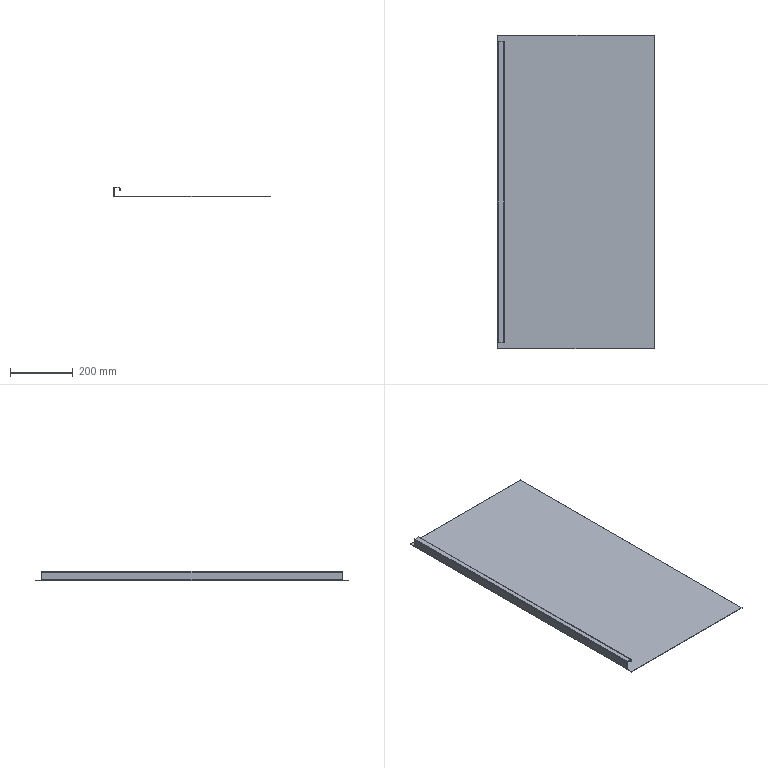Component | SolidWorks | BottomPlate-2 | 1 solid | 38 faces | box 500 x 1000 x 30 mm | volume 826993 mm3 | plane 32 | cylinder 6 | commonest cylinder face diameters 4.473 x2 1.473 x2 5 x1 2 x1
STEP:
#1=CARTESIAN_POINT('',(0.6403,28.583,-3.996));
#2=VERTEX_POINT('',#1);
#3=CARTESIAN_POINT('',(0.6403,28.583,-3.937));
#4=VERTEX_POINT('',#3);
#5=CARTESIAN_POINT('',(0.6403,28.583,-3.996));
#6=DIRECTION('',(0.,0.,1.));
#7=VECTOR('',#6,39.37);
#8=LINE('',#5,#7);
#9=EDGE_CURVE('',#2,#4,#8,.T.);
#10=ORIENTED_EDGE('',*,*,#9,.F.);
#11=CARTESIAN_POINT('',(0.029,28.583,-3.996));
#12=VERTEX_POINT('',#11);
#13=CARTESIAN_POINT('',(-0.,28.583,-3.996));
#14=DIRECTION('',(-1.,-0.,0.));
#15=VECTOR('',#14,39.37);
#16=LINE('',#13,#15);
#17=EDGE_CURVE('',#2,#12,#16,.T.);
#18=ORIENTED_EDGE('',*,*,#17,.T.);
#19=CARTESIAN_POINT('',(0.029,28.583,-3.937));
#20=VERTEX_POINT('',#19);
#21=CARTESIAN_POINT('',(0.029,28.583,-3.937));
#22=DIRECTION('',(0.,-0.,1.));
#23=VECTOR('',#22,39.37);
#24=LINE('',#21,#23);
#25=EDGE_CURVE('',#12,#20,#24,.T.);
#26=ORIENTED_EDGE('',*,*,#25,.T.);
#27=CARTESIAN_POINT('',(9.783,28.583,-3.937));
#28=DIRECTION('',(-1.,-0.,0.));
#29=VECTOR('',#28,39.37);
#30=LINE('',#27,#29);
#31=EDGE_CURVE('',#4,#20,#30,.T.);
#32=ORIENTED_EDGE('',*,*,#31,.F.);
#33=EDGE_LOOP('',(#10,#18,#26,#32));
#34=FACE_OUTER_BOUND('',#33,.T.);
#35=CARTESIAN_POINT('',(-0.,28.583,-3.937));
#36=DIRECTION('',(0.,-1.,-0.));
#37=DIRECTION('',(0.,-0.,1.));
#38=AXIS2_PLACEMENT_3D('',#35,#36,#37);
#39=PLANE('',#38);
#40=ADVANCED_FACE('',(#34),#39,.F.);
#41=CARTESIAN_POINT('',(0.6403,-9.213,-3.996));
#42=VERTEX_POINT('',#41);
#43=CARTESIAN_POINT('',(0.6403,-9.213,-3.937));
#44=VERTEX_POINT('',#43);
#45=CARTESIAN_POINT('',(0.6403,-9.213,-3.996));
#46=DIRECTION('',(0.,-0.,1.));
#47=VECTOR('',#46,39.37);
#48=LINE('',#45,#47);
#49=EDGE_CURVE('',#42,#44,#48,.T.);
#50=ORIENTED_EDGE('',*,*,#49,.T.);
#51=CARTESIAN_POINT('',(0.029,-9.213,-3.937));
#52=VERTEX_POINT('',#51);
#53=CARTESIAN_POINT('',(9.783,-9.213,-3.937));
#54=DIRECTION('',(1.,0.,-0.));
#55=VECTOR('',#54,39.37);
#56=LINE('',#53,#55);
#57=EDGE_CURVE('',#52,#44,#56,.T.);
#58=ORIENTED_EDGE('',*,*,#57,.F.);
#59=CARTESIAN_POINT('',(0.029,-9.213,-3.996));
#60=VERTEX_POINT('',#59);
#61=CARTESIAN_POINT('',(0.029,-9.213,-3.996));
#62=DIRECTION('',(0.,-0.,1.));
#63=VECTOR('',#62,39.37);
#64=LINE('',#61,#63);
#65=EDGE_CURVE('',#60,#52,#64,.T.);
#66=ORIENTED_EDGE('',*,*,#65,.F.);
#67=CARTESIAN_POINT('',(0.7283,-9.213,-3.996));
#68=DIRECTION('',(1.,0.,-0.));
#69=VECTOR('',#68,39.37);
#70=LINE('',#67,#69);
#71=EDGE_CURVE('',#60,#42,#70,.T.);
#72=ORIENTED_EDGE('',*,*,#71,.T.);
#73=EDGE_LOOP('',(#50,#58,#66,#72));
#74=FACE_OUTER_BOUND('',#73,.T.);
#75=CARTESIAN_POINT('',(0.7283,-9.213,-3.937));
#76=DIRECTION('',(-0.,1.,0.));
#77=DIRECTION('',(-0.,0.,-1.));
#78=AXIS2_PLACEMENT_3D('',#75,#76,#77);
#79=PLANE('',#78);
#80=ADVANCED_FACE('',(#74),#79,.F.);
#81=CARTESIAN_POINT('',(0.6403,-9.213,-3.937));
#82=DIRECTION('',(-0.,1.,0.));
#83=VECTOR('',#82,39.37);
#84=LINE('',#81,#83);
#85=EDGE_CURVE('',#44,#4,#84,.T.);
#86=ORIENTED_EDGE('',*,*,#85,.T.);
#87=ORIENTED_EDGE('',*,*,#31,.T.);
#88=CARTESIAN_POINT('',(0.029,28.583,-3.937));
#89=DIRECTION('',(-0.,1.,0.));
#90=VECTOR('',#89,39.37);
#91=LINE('',#88,#90);
#92=EDGE_CURVE('',#52,#20,#91,.T.);
#93=ORIENTED_EDGE('',*,*,#92,.F.);
#94=ORIENTED_EDGE('',*,*,#57,.T.);
#95=EDGE_LOOP('',(#86,#87,#93,#94));
#96=FACE_OUTER_BOUND('',#95,.T.);
#97=CARTESIAN_POINT('',(9.783,9.685,-3.937));
#98=DIRECTION('',(-0.,0.,-1.));
#99=DIRECTION('',(-1.,-0.,0.));
#100=AXIS2_PLACEMENT_3D('',#97,#98,#99);
#101=PLANE('',#100);
#102=ADVANCED_FACE('',(#96),#101,.F.);
#103=ORIENTED_EDGE('',*,*,#17,.F.);
#104=CARTESIAN_POINT('',(0.6403,-9.213,-3.996));
#105=DIRECTION('',(-0.,1.,0.));
#106=VECTOR('',#105,39.37);
#107=LINE('',#104,#106);
#108=EDGE_CURVE('',#42,#2,#107,.T.);
#109=ORIENTED_EDGE('',*,*,#108,.F.);
#110=ORIENTED_EDGE('',*,*,#71,.F.);
#111=CARTESIAN_POINT('',(0.029,28.583,-3.996));
#112=DIRECTION('',(0.,-1.,-0.));
#113=VECTOR('',#112,39.37);
#114=LINE('',#111,#113);
#115=EDGE_CURVE('',#12,#60,#114,.T.);
#116=ORIENTED_EDGE('',*,*,#115,.F.);
#117=EDGE_LOOP('',(#103,#109,#110,#116));
#118=FACE_OUTER_BOUND('',#117,.T.);
#119=CARTESIAN_POINT('',(9.783,9.685,-3.996));
#120=DIRECTION('',(-0.,0.,-1.));
#121=DIRECTION('',(-1.,-0.,0.));
#122=AXIS2_PLACEMENT_3D('',#119,#120,#121);
#123=PLANE('',#122);
#124=ADVANCED_FACE('',(#118),#123,.T.);
#125=CARTESIAN_POINT('',(0.,-9.213,-4.025));
#126=VERTEX_POINT('',#125);
#127=CARTESIAN_POINT('',(0.,-9.213,-5.02));
#128=VERTEX_POINT('',#127);
#129=CARTESIAN_POINT('',(0.,-9.213,-5.118));
#130=DIRECTION('',(-0.,-0.,-1.));
#131=VECTOR('',#130,39.37);
#132=LINE('',#129,#131);
#133=EDGE_CURVE('',#126,#128,#132,.T.);
#134=ORIENTED_EDGE('',*,*,#133,.F.);
#135=CARTESIAN_POINT('',(-0.05906,-9.213,-4.025));
#136=VERTEX_POINT('',#135);
#137=CARTESIAN_POINT('',(0.,-9.213,-4.025));
#138=DIRECTION('',(-1.,-0.,-0.));
#139=VECTOR('',#138,39.37);
#140=LINE('',#137,#139);
#141=EDGE_CURVE('',#126,#136,#140,.T.);
#142=ORIENTED_EDGE('',*,*,#141,.T.);
#143=CARTESIAN_POINT('',(-0.05906,-9.213,-5.02));
#144=VERTEX_POINT('',#143);
#145=CARTESIAN_POINT('',(-0.05906,-9.213,-3.937));
#146=DIRECTION('',(-0.,-0.,-1.));
#147=VECTOR('',#146,39.37);
#148=LINE('',#145,#147);
#149=EDGE_CURVE('',#136,#144,#148,.T.);
#150=ORIENTED_EDGE('',*,*,#149,.T.);
#151=CARTESIAN_POINT('',(0.,-9.213,-5.02));
#152=DIRECTION('',(-1.,-0.,0.));
#153=VECTOR('',#152,39.37);
#154=LINE('',#151,#153);
#155=EDGE_CURVE('',#128,#144,#154,.T.);
#156=ORIENTED_EDGE('',*,*,#155,.F.);
#157=EDGE_LOOP('',(#134,#142,#150,#156));
#158=FACE_OUTER_BOUND('',#157,.T.);
#159=CARTESIAN_POINT('',(-0.05906,-9.213,-3.937));
#160=DIRECTION('',(0.,-1.,0.));
#161=DIRECTION('',(-1.,-0.,0.));
#162=AXIS2_PLACEMENT_3D('',#159,#160,#161);
#163=PLANE('',#162);
#164=ADVANCED_FACE('',(#158),#163,.T.);
#165=CARTESIAN_POINT('',(-0.05906,28.583,-4.025));
#166=VERTEX_POINT('',#165);
#167=CARTESIAN_POINT('',(-0.05906,-9.213,-4.025));
#168=DIRECTION('',(-0.,1.,-0.));
#169=VECTOR('',#168,39.37);
#170=LINE('',#167,#169);
#171=EDGE_CURVE('',#136,#166,#170,.T.);
#172=ORIENTED_EDGE('',*,*,#171,.T.);
#173=CARTESIAN_POINT('',(-0.05906,28.583,-5.02));
#174=VERTEX_POINT('',#173);
#175=CARTESIAN_POINT('',(-0.05906,28.583,-5.059));
#176=DIRECTION('',(0.,0.,1.));
#177=VECTOR('',#176,39.37);
#178=LINE('',#175,#177);
#179=EDGE_CURVE('',#174,#166,#178,.T.);
#180=ORIENTED_EDGE('',*,*,#179,.F.);
#181=CARTESIAN_POINT('',(-0.05906,28.583,-5.02));
#182=DIRECTION('',(-0.,1.,-0.));
#183=VECTOR('',#182,39.37);
#184=LINE('',#181,#183);
#185=EDGE_CURVE('',#144,#174,#184,.T.);
#186=ORIENTED_EDGE('',*,*,#185,.F.);
#187=ORIENTED_EDGE('',*,*,#149,.F.);
#188=EDGE_LOOP('',(#172,#180,#186,#187));
#189=FACE_OUTER_BOUND('',#188,.T.);
#190=CARTESIAN_POINT('',(-0.05906,9.685,-5.118));
#191=DIRECTION('',(1.,0.,-0.));
#192=DIRECTION('',(-0.,-0.,-1.));
#193=AXIS2_PLACEMENT_3D('',#190,#191,#192);
#194=PLANE('',#193);
#195=ADVANCED_FACE('',(#189),#194,.F.);
#196=CARTESIAN_POINT('',(-0.,28.583,-5.02));
#197=VERTEX_POINT('',#196);
#198=CARTESIAN_POINT('',(-0.,28.583,-4.025));
#199=VERTEX_POINT('',#198);
#200=CARTESIAN_POINT('',(-0.,28.583,-5.118));
#201=DIRECTION('',(0.,0.,1.));
#202=VECTOR('',#201,39.37);
#203=LINE('',#200,#202);
#204=EDGE_CURVE('',#197,#199,#203,.T.);
#205=ORIENTED_EDGE('',*,*,#204,.T.);
#206=CARTESIAN_POINT('',(0.,-9.213,-4.025));
#207=DIRECTION('',(-0.,1.,-0.));
#208=VECTOR('',#207,39.37);
#209=LINE('',#206,#208);
#210=EDGE_CURVE('',#126,#199,#209,.T.);
#211=ORIENTED_EDGE('',*,*,#210,.F.);
#212=ORIENTED_EDGE('',*,*,#133,.T.);
#213=CARTESIAN_POINT('',(-0.,28.583,-5.02));
#214=DIRECTION('',(0.,-1.,0.));
#215=VECTOR('',#214,39.37);
#216=LINE('',#213,#215);
#217=EDGE_CURVE('',#197,#128,#216,.T.);
#218=ORIENTED_EDGE('',*,*,#217,.F.);
#219=EDGE_LOOP('',(#205,#211,#212,#218));
#220=FACE_OUTER_BOUND('',#219,.T.);
#221=CARTESIAN_POINT('',(-0.,9.685,-5.118));
#222=DIRECTION('',(1.,0.,-0.));
#223=DIRECTION('',(-0.,-0.,-1.));
#224=AXIS2_PLACEMENT_3D('',#221,#222,#223);
#225=PLANE('',#224);
#226=ADVANCED_FACE('',(#220),#225,.T.);
#227=CARTESIAN_POINT('',(-0.05906,-10.,-5.059));
#228=VERTEX_POINT('',#227);
#229=CARTESIAN_POINT('',(-0.05906,-9.242,-5.059));
#230=VERTEX_POINT('',#229);
#231=CARTESIAN_POINT('',(-0.05906,-10.,-5.059));
#232=DIRECTION('',(-0.,1.,-0.));
#233=VECTOR('',#232,39.37);
#234=LINE('',#231,#233);
#235=EDGE_CURVE('',#228,#230,#234,.T.);
#236=ORIENTED_EDGE('',*,*,#235,.T.);
#237=CARTESIAN_POINT('',(-0.05906,-9.242,-5.118));
#238=VERTEX_POINT('',#237);
#239=CARTESIAN_POINT('',(-0.05906,-9.242,-5.059));
#240=DIRECTION('',(-0.,-0.,-1.));
#241=VECTOR('',#240,39.37);
#242=LINE('',#239,#241);
#243=EDGE_CURVE('',#230,#238,#242,.T.);
#244=ORIENTED_EDGE('',*,*,#243,.T.);
#245=CARTESIAN_POINT('',(-0.05906,-10.,-5.118));
#246=VERTEX_POINT('',#245);
#247=CARTESIAN_POINT('',(-0.05906,-10.,-5.118));
#248=DIRECTION('',(-0.,1.,-0.));
#249=VECTOR('',#248,39.37);
#250=LINE('',#247,#249);
#251=EDGE_CURVE('',#246,#238,#250,.T.);
#252=ORIENTED_EDGE('',*,*,#251,.F.);
#253=CARTESIAN_POINT('',(-0.05906,-10.,-5.059));
#254=DIRECTION('',(-0.,-0.,-1.));
#255=VECTOR('',#254,39.37);
#256=LINE('',#253,#255);
#257=EDGE_CURVE('',#228,#246,#256,.T.);
#258=ORIENTED_EDGE('',*,*,#257,.F.);
#259=EDGE_LOOP('',(#236,#244,#252,#258));
#260=FACE_OUTER_BOUND('',#259,.T.);
#261=CARTESIAN_POINT('',(-0.05906,-10.,-5.059));
#262=DIRECTION('',(-1.,-0.,0.));
#263=DIRECTION('',(-0.,1.,-0.));
#264=AXIS2_PLACEMENT_3D('',#261,#262,#263);
#265=PLANE('',#264);
#266=ADVANCED_FACE('',(#260),#265,.T.);
#267=CARTESIAN_POINT('',(-0.05906,28.612,-5.118));
#268=VERTEX_POINT('',#267);
#269=CARTESIAN_POINT('',(-0.05906,29.37,-5.118));
#270=VERTEX_POINT('',#269);
#271=CARTESIAN_POINT('',(-0.05906,-10.,-5.118));
#272=DIRECTION('',(-0.,1.,-0.));
#273=VECTOR('',#272,39.37);
#274=LINE('',#271,#273);
#275=EDGE_CURVE('',#268,#270,#274,.T.);
#276=ORIENTED_EDGE('',*,*,#275,.F.);
#277=CARTESIAN_POINT('',(-0.05906,28.612,-5.059));
#278=VERTEX_POINT('',#277);
#279=CARTESIAN_POINT('',(-0.05906,28.612,-5.059));
#280=DIRECTION('',(-0.,-0.,-1.));
#281=VECTOR('',#280,39.37);
#282=LINE('',#279,#281);
#283=EDGE_CURVE('',#278,#268,#282,.T.);
#284=ORIENTED_EDGE('',*,*,#283,.F.);
#285=CARTESIAN_POINT('',(-0.05906,29.37,-5.059));
#286=VERTEX_POINT('',#285);
#287=CARTESIAN_POINT('',(-0.05906,-10.,-5.059));
#288=DIRECTION('',(-0.,1.,-0.));
#289=VECTOR('',#288,39.37);
#290=LINE('',#287,#289);
#291=EDGE_CURVE('',#278,#286,#290,.T.);
#292=ORIENTED_EDGE('',*,*,#291,.T.);
#293=CARTESIAN_POINT('',(-0.05906,29.37,-5.059));
#294=DIRECTION('',(-0.,-0.,-1.));
#295=VECTOR('',#294,39.37);
#296=LINE('',#293,#295);
#297=EDGE_CURVE('',#286,#270,#296,.T.);
#298=ORIENTED_EDGE('',*,*,#297,.T.);
#299=EDGE_LOOP('',(#276,#284,#292,#298));
#300=FACE_OUTER_BOUND('',#299,.T.);
#301=CARTESIAN_POINT('',(-0.05906,-10.,-5.059));
#302=DIRECTION('',(-1.,-0.,0.));
#303=DIRECTION('',(-0.,1.,-0.));
#304=AXIS2_PLACEMENT_3D('',#301,#302,#303);
#305=PLANE('',#304);
#306=ADVANCED_FACE('',(#300),#305,.T.);
#307=CARTESIAN_POINT('',(0.0689,-9.242,-5.059));
#308=VERTEX_POINT('',#307);
#309=CARTESIAN_POINT('',(-0.05906,-9.242,-5.059));
#310=DIRECTION('',(1.,0.,-0.));
#311=VECTOR('',#310,39.37);
#312=LINE('',#309,#311);
#313=EDGE_CURVE('',#230,#308,#312,.T.);
#314=ORIENTED_EDGE('',*,*,#313,.F.);
#315=ORIENTED_EDGE('',*,*,#235,.F.);
#316=CARTESIAN_POINT('',(19.626,-10.,-5.059));
#317=VERTEX_POINT('',#316);
#318=CARTESIAN_POINT('',(19.626,-10.,-5.059));
#319=DIRECTION('',(-1.,-0.,0.));
#320=VECTOR('',#319,39.37);
#321=LINE('',#318,#320);
#322=EDGE_CURVE('',#317,#228,#321,.T.);
#323=ORIENTED_EDGE('',*,*,#322,.F.);
#324=CARTESIAN_POINT('',(19.626,29.37,-5.059));
#325=VERTEX_POINT('',#324);
#326=CARTESIAN_POINT('',(19.626,-10.,-5.059));
#327=DIRECTION('',(0.,-1.,0.));
#328=VECTOR('',#327,39.37);
#329=LINE('',#326,#328);
#330=EDGE_CURVE('',#325,#317,#329,.T.);
#331=ORIENTED_EDGE('',*,*,#330,.F.);
#332=CARTESIAN_POINT('',(19.626,29.37,-5.059));
#333=DIRECTION('',(1.,0.,-0.));
#334=VECTOR('',#333,39.37);
#335=LINE('',#332,#334);
#336=EDGE_CURVE('',#286,#325,#335,.T.);
#337=ORIENTED_EDGE('',*,*,#336,.F.);
#338=ORIENTED_EDGE('',*,*,#291,.F.);
#339=CARTESIAN_POINT('',(0.0689,28.612,-5.059));
#340=VERTEX_POINT('',#339);
#341=CARTESIAN_POINT('',(0.0689,28.612,-5.059));
#342=DIRECTION('',(-1.,0.,0.));
#343=VECTOR('',#342,39.37);
#344=LINE('',#341,#343);
#345=EDGE_CURVE('',#340,#278,#344,.T.);
#346=ORIENTED_EDGE('',*,*,#345,.F.);
#347=CARTESIAN_POINT('',(0.0689,28.583,-5.059));
#348=VERTEX_POINT('',#347);
#349=CARTESIAN_POINT('',(0.0689,28.583,-5.059));
#350=DIRECTION('',(-0.,1.,-0.));
#351=VECTOR('',#350,39.37);
#352=LINE('',#349,#351);
#353=EDGE_CURVE('',#348,#340,#352,.T.);
#354=ORIENTED_EDGE('',*,*,#353,.F.);
#355=CARTESIAN_POINT('',(0.03937,28.583,-5.059));
#356=VERTEX_POINT('',#355);
#357=CARTESIAN_POINT('',(0.03937,28.583,-5.059));
#358=DIRECTION('',(1.,0.,-0.));
#359=VECTOR('',#358,39.37);
#360=LINE('',#357,#359);
#361=EDGE_CURVE('',#356,#348,#360,.T.);
#362=ORIENTED_EDGE('',*,*,#361,.F.);
#363=CARTESIAN_POINT('',(0.03937,-9.213,-5.059));
#364=VERTEX_POINT('',#363);
#365=CARTESIAN_POINT('',(0.03937,-9.213,-5.059));
#366=DIRECTION('',(-0.,1.,-0.));
#367=VECTOR('',#366,39.37);
#368=LINE('',#365,#367);
#369=EDGE_CURVE('',#364,#356,#368,.T.);
#370=ORIENTED_EDGE('',*,*,#369,.F.);
#371=CARTESIAN_POINT('',(0.0689,-9.213,-5.059));
#372=VERTEX_POINT('',#371);
#373=CARTESIAN_POINT('',(0.0689,-9.213,-5.059));
#374=DIRECTION('',(-1.,-0.,0.));
#375=VECTOR('',#374,39.37);
#376=LINE('',#373,#375);
#377=EDGE_CURVE('',#372,#364,#376,.T.);
#378=ORIENTED_EDGE('',*,*,#377,.F.);
#379=CARTESIAN_POINT('',(0.0689,-9.242,-5.059));
#380=DIRECTION('',(-0.,1.,-0.));
#381=VECTOR('',#380,39.37);
#382=LINE('',#379,#381);
#383=EDGE_CURVE('',#308,#372,#382,.T.);
#384=ORIENTED_EDGE('',*,*,#383,.F.);
#385=EDGE_LOOP('',(#314,#315,#323,#331,#337,#338,#346,#354,#362,#370,#378,#384));
#386=FACE_OUTER_BOUND('',#385,.T.);
#387=CARTESIAN_POINT('',(9.783,9.685,-5.059));
#388=DIRECTION('',(-0.,-0.,-1.));
#389=DIRECTION('',(-1.,-0.,0.));
#390=AXIS2_PLACEMENT_3D('',#387,#388,#389);
#391=PLANE('',#390);
#392=ADVANCED_FACE('',(#386),#391,.F.);
#393=ORIENTED_EDGE('',*,*,#251,.T.);
#394=CARTESIAN_POINT('',(0.0689,-9.242,-5.118));
#395=VERTEX_POINT('',#394);
#396=CARTESIAN_POINT('',(9.783,-9.242,-5.118));
#397=DIRECTION('',(1.,0.,-0.));
#398=VECTOR('',#397,39.37);
#399=LINE('',#396,#398);
#400=EDGE_CURVE('',#238,#395,#399,.T.);
#401=ORIENTED_EDGE('',*,*,#400,.T.);
#402=CARTESIAN_POINT('',(0.0689,-9.213,-5.118));
#403=VERTEX_POINT('',#402);
#404=CARTESIAN_POINT('',(0.0689,9.685,-5.118));
#405=DIRECTION('',(-0.,1.,-0.));
#406=VECTOR('',#405,39.37);
#407=LINE('',#404,#406);
#408=EDGE_CURVE('',#395,#403,#407,.T.);
#409=ORIENTED_EDGE('',*,*,#408,.T.);
#410=CARTESIAN_POINT('',(0.03937,-9.213,-5.118));
#411=VERTEX_POINT('',#410);
#412=CARTESIAN_POINT('',(9.783,-9.213,-5.118));
#413=DIRECTION('',(-1.,-0.,0.));
#414=VECTOR('',#413,39.37);
#415=LINE('',#412,#414);
#416=EDGE_CURVE('',#403,#411,#415,.T.);
#417=ORIENTED_EDGE('',*,*,#416,.T.);
#418=CARTESIAN_POINT('',(0.03937,28.583,-5.118));
#419=VERTEX_POINT('',#418);
#420=CARTESIAN_POINT('',(0.03937,-9.213,-5.118));
#421=DIRECTION('',(-0.,1.,-0.));
#422=VECTOR('',#421,39.37);
#423=LINE('',#420,#422);
#424=EDGE_CURVE('',#411,#419,#423,.T.);
#425=ORIENTED_EDGE('',*,*,#424,.T.);
#426=CARTESIAN_POINT('',(0.0689,28.583,-5.118));
#427=VERTEX_POINT('',#426);
#428=CARTESIAN_POINT('',(9.783,28.583,-5.118));
#429=DIRECTION('',(1.,0.,-0.));
#430=VECTOR('',#429,39.37);
#431=LINE('',#428,#430);
#432=EDGE_CURVE('',#419,#427,#431,.T.);
#433=ORIENTED_EDGE('',*,*,#432,.T.);
#434=CARTESIAN_POINT('',(0.0689,28.612,-5.118));
#435=VERTEX_POINT('',#434);
#436=CARTESIAN_POINT('',(0.0689,9.685,-5.118));
#437=DIRECTION('',(-0.,1.,-0.));
#438=VECTOR('',#437,39.37);
#439=LINE('',#436,#438);
#440=EDGE_CURVE('',#427,#435,#439,.T.);
#441=ORIENTED_EDGE('',*,*,#440,.T.);
#442=CARTESIAN_POINT('',(9.783,28.612,-5.118));
#443=DIRECTION('',(-1.,0.,0.));
#444=VECTOR('',#443,39.37);
#445=LINE('',#442,#444);
#446=EDGE_CURVE('',#435,#268,#445,.T.);
#447=ORIENTED_EDGE('',*,*,#446,.T.);
#448=ORIENTED_EDGE('',*,*,#275,.T.);
#449=CARTESIAN_POINT('',(19.626,29.37,-5.118));
#450=VERTEX_POINT('',#449);
#451=CARTESIAN_POINT('',(19.626,29.37,-5.118));
#452=DIRECTION('',(1.,0.,-0.));
#453=VECTOR('',#452,39.37);
#454=LINE('',#451,#453);
#455=EDGE_CURVE('',#270,#450,#454,.T.);
#456=ORIENTED_EDGE('',*,*,#455,.T.);
#457=CARTESIAN_POINT('',(19.626,-10.,-5.118));
#458=VERTEX_POINT('',#457);
#459=CARTESIAN_POINT('',(19.626,-10.,-5.118));
#460=DIRECTION('',(0.,-1.,0.));
#461=VECTOR('',#460,39.37);
#462=LINE('',#459,#461);
#463=EDGE_CURVE('',#450,#458,#462,.T.);
#464=ORIENTED_EDGE('',*,*,#463,.T.);
#465=CARTESIAN_POINT('',(19.626,-10.,-5.118));
#466=DIRECTION('',(-1.,-0.,0.));
#467=VECTOR('',#466,39.37);
#468=LINE('',#465,#467);
#469=EDGE_CURVE('',#458,#246,#468,.T.);
#470=ORIENTED_EDGE('',*,*,#469,.T.);
#471=EDGE_LOOP('',(#393,#401,#409,#417,#425,#433,#441,#447,#448,#456,#464,#470));
#472=FACE_OUTER_BOUND('',#471,.T.);
#473=CARTESIAN_POINT('',(9.783,9.685,-5.118));
#474=DIRECTION('',(-0.,-0.,-1.));
#475=DIRECTION('',(-1.,-0.,0.));
#476=AXIS2_PLACEMENT_3D('',#473,#474,#475);
#477=PLANE('',#476);
#478=ADVANCED_FACE('',(#472),#477,.T.);
#479=ORIENTED_EDGE('',*,*,#455,.F.);
#480=ORIENTED_EDGE('',*,*,#297,.F.);
#481=ORIENTED_EDGE('',*,*,#336,.T.);
#482=CARTESIAN_POINT('',(19.626,29.37,-5.059));
#483=DIRECTION('',(-0.,-0.,-1.));
#484=VECTOR('',#483,39.37);
#485=LINE('',#482,#484);
#486=EDGE_CURVE('',#325,#450,#485,.T.);
#487=ORIENTED_EDGE('',*,*,#486,.T.);
#488=EDGE_LOOP('',(#479,#480,#481,#487));
#489=FACE_OUTER_BOUND('',#488,.T.);
#490=CARTESIAN_POINT('',(19.626,29.37,-5.059));
#491=DIRECTION('',(-0.,1.,-0.));
#492=DIRECTION('',(1.,0.,-0.));
#493=AXIS2_PLACEMENT_3D('',#490,#491,#492);
#494=PLANE('',#493);
#495=ADVANCED_FACE('',(#489),#494,.T.);
#496=ORIENTED_EDGE('',*,*,#469,.F.);
#497=CARTESIAN_POINT('',(19.626,-10.,-5.059));
#498=DIRECTION('',(-0.,-0.,-1.));
#499=VECTOR('',#498,39.37);
#500=LINE('',#497,#499);
#501=EDGE_CURVE('',#317,#458,#500,.T.);
#502=ORIENTED_EDGE('',*,*,#501,.F.);
#503=ORIENTED_EDGE('',*,*,#322,.T.);
#504=ORIENTED_EDGE('',*,*,#257,.T.);
#505=EDGE_LOOP('',(#496,#502,#503,#504));
#506=FACE_OUTER_BOUND('',#505,.T.);
#507=CARTESIAN_POINT('',(19.626,-10.,-5.059));
#508=DIRECTION('',(0.,-1.,0.));
#509=DIRECTION('',(-1.,-0.,0.));
#510=AXIS2_PLACEMENT_3D('',#507,#508,#509);
#511=PLANE('',#510);
#512=ADVANCED_FACE('',(#506),#511,.T.);
#513=ORIENTED_EDGE('',*,*,#463,.F.);
#514=ORIENTED_EDGE('',*,*,#486,.F.);
#515=ORIENTED_EDGE('',*,*,#330,.T.);
#516=ORIENTED_EDGE('',*,*,#501,.T.);
#517=EDGE_LOOP('',(#513,#514,#515,#516));
#518=FACE_OUTER_BOUND('',#517,.T.);
#519=CARTESIAN_POINT('',(19.626,-10.,-5.059));
#520=DIRECTION('',(1.,0.,-0.));
#521=DIRECTION('',(0.,-1.,0.));
#522=AXIS2_PLACEMENT_3D('',#519,#520,#521);
#523=PLANE('',#522);
#524=ADVANCED_FACE('',(#518),#523,.T.);
#525=ORIENTED_EDGE('',*,*,#400,.F.);
#526=ORIENTED_EDGE('',*,*,#243,.F.);
#527=ORIENTED_EDGE('',*,*,#313,.T.);
#528=CARTESIAN_POINT('',(0.0689,-9.242,-5.059));
#529=DIRECTION('',(-0.,-0.,-1.));
#530=VECTOR('',#529,39.37);
#531=LINE('',#528,#530);
#532=EDGE_CURVE('',#308,#395,#531,.T.);
#533=ORIENTED_EDGE('',*,*,#532,.T.);
#534=EDGE_LOOP('',(#525,#526,#527,#533));
#535=FACE_OUTER_BOUND('',#534,.T.);
#536=CARTESIAN_POINT('',(-0.05906,-9.242,-5.059));
#537=DIRECTION('',(-0.,1.,-0.));
#538=DIRECTION('',(1.,0.,-0.));
#539=AXIS2_PLACEMENT_3D('',#536,#537,#538);
#540=PLANE('',#539);
#541=ADVANCED_FACE('',(#535),#540,.T.);
#542=ORIENTED_EDGE('',*,*,#408,.F.);
#543=ORIENTED_EDGE('',*,*,#532,.F.);
#544=ORIENTED_EDGE('',*,*,#383,.T.);
#545=CARTESIAN_POINT('',(0.0689,-9.213,-5.059));
#546=DIRECTION('',(-0.,-0.,-1.));
#547=VECTOR('',#546,39.37);
#548=LINE('',#545,#547);
#549=EDGE_CURVE('',#372,#403,#548,.T.);
#550=ORIENTED_EDGE('',*,*,#549,.T.);
#551=EDGE_LOOP('',(#542,#543,#544,#550));
#552=FACE_OUTER_BOUND('',#551,.T.);
#553=CARTESIAN_POINT('',(0.0689,-9.242,-5.059));
#554=DIRECTION('',(-1.,-0.,0.));
#555=DIRECTION('',(0.,0.,1.));
#556=AXIS2_PLACEMENT_3D('',#553,#554,#555);
#557=PLANE('',#556);
#558=ADVANCED_FACE('',(#552),#557,.T.);
#559=ORIENTED_EDGE('',*,*,#416,.F.);
#560=ORIENTED_EDGE('',*,*,#549,.F.);
#561=ORIENTED_EDGE('',*,*,#377,.T.);
#562=CARTESIAN_POINT('',(0.03937,-9.213,-5.059));
#563=DIRECTION('',(-0.,-0.,-1.));
#564=VECTOR('',#563,39.37);
#565=LINE('',#562,#564);
#566=EDGE_CURVE('',#364,#411,#565,.T.);
#567=ORIENTED_EDGE('',*,*,#566,.T.);
#568=EDGE_LOOP('',(#559,#560,#561,#567));
#569=FACE_OUTER_BOUND('',#568,.T.);
#570=CARTESIAN_POINT('',(0.0689,-9.213,-5.059));
#571=DIRECTION('',(0.,-1.,0.));
#572=DIRECTION('',(-1.,-0.,0.));
#573=AXIS2_PLACEMENT_3D('',#570,#571,#572);
#574=PLANE('',#573);
#575=ADVANCED_FACE('',(#569),#574,.T.);
#576=ORIENTED_EDGE('',*,*,#432,.F.);
#577=CARTESIAN_POINT('',(0.03937,28.583,-5.059));
#578=DIRECTION('',(-0.,-0.,-1.));
#579=VECTOR('',#578,39.37);
#580=LINE('',#577,#579);
#581=EDGE_CURVE('',#356,#419,#580,.T.);
#582=ORIENTED_EDGE('',*,*,#581,.F.);
#583=ORIENTED_EDGE('',*,*,#361,.T.);
#584=CARTESIAN_POINT('',(0.0689,28.583,-5.059));
#585=DIRECTION('',(-0.,-0.,-1.));
#586=VECTOR('',#585,39.37);
#587=LINE('',#584,#586);
#588=EDGE_CURVE('',#348,#427,#587,.T.);
#589=ORIENTED_EDGE('',*,*,#588,.T.);
#590=EDGE_LOOP('',(#576,#582,#583,#589));
#591=FACE_OUTER_BOUND('',#590,.T.);
#592=CARTESIAN_POINT('',(0.03937,28.583,-5.059));
#593=DIRECTION('',(-0.,1.,-0.));
#594=DIRECTION('',(1.,0.,-0.));
#595=AXIS2_PLACEMENT_3D('',#592,#593,#594);
#596=PLANE('',#595);
#597=ADVANCED_FACE('',(#591),#596,.T.);
#598=ORIENTED_EDGE('',*,*,#440,.F.);
#599=ORIENTED_EDGE('',*,*,#588,.F.);
#600=ORIENTED_EDGE('',*,*,#353,.T.);
#601=CARTESIAN_POINT('',(0.0689,28.612,-5.059));
#602=DIRECTION('',(-0.,-0.,-1.));
#603=VECTOR('',#602,39.37);
#604=LINE('',#601,#603);
#605=EDGE_CURVE('',#340,#435,#604,.T.);
#606=ORIENTED_EDGE('',*,*,#605,.T.);
#607=EDGE_LOOP('',(#598,#599,#600,#606));
#608=FACE_OUTER_BOUND('',#607,.T.);
#609=CARTESIAN_POINT('',(0.0689,28.583,-5.059));
#610=DIRECTION('',(-1.,-0.,0.));
#611=DIRECTION('',(0.,0.,1.));
#612=AXIS2_PLACEMENT_3D('',#609,#610,#611);
#613=PLANE('',#612);
#614=ADVANCED_FACE('',(#608),#613,.T.);
#615=ORIENTED_EDGE('',*,*,#446,.F.);
#616=ORIENTED_EDGE('',*,*,#605,.F.);
#617=ORIENTED_EDGE('',*,*,#345,.T.);
#618=ORIENTED_EDGE('',*,*,#283,.T.);
#619=EDGE_LOOP('',(#615,#616,#617,#618));
#620=FACE_OUTER_BOUND('',#619,.T.);
#621=CARTESIAN_POINT('',(0.0689,28.612,-5.059));
#622=DIRECTION('',(-0.,-1.,0.));
#623=DIRECTION('',(-1.,0.,0.));
#624=AXIS2_PLACEMENT_3D('',#621,#622,#623);
#625=PLANE('',#624);
#626=ADVANCED_FACE('',(#620),#625,.T.);
#627=CARTESIAN_POINT('',(-0.05906,28.583,-5.02));
#628=DIRECTION('',(-1.,-0.,0.));
#629=VECTOR('',#628,39.37);
#630=LINE('',#627,#629);
#631=EDGE_CURVE('',#197,#174,#630,.T.);
#632=ORIENTED_EDGE('',*,*,#631,.F.);
#633=CARTESIAN_POINT('',(0.03937,28.583,-5.02));
#634=DIRECTION('',(-0.,1.,-0.));
#635=DIRECTION('',(-1.,0.,0.));
#636=AXIS2_PLACEMENT_3D('',#633,#634,#635);
#637=CIRCLE('',#636,0.03937);
#638=EDGE_CURVE('',#356,#197,#637,.T.);
#639=ORIENTED_EDGE('',*,*,#638,.F.);
#640=ORIENTED_EDGE('',*,*,#581,.T.);
#641=CARTESIAN_POINT('',(0.03937,28.583,-5.02));
#642=DIRECTION('',(-0.,1.,-0.));
#643=DIRECTION('',(-1.,0.,0.));
#644=AXIS2_PLACEMENT_3D('',#641,#642,#643);
#645=CIRCLE('',#644,0.09843);
#646=EDGE_CURVE('',#419,#174,#645,.T.);
#647=ORIENTED_EDGE('',*,*,#646,.T.);
#648=EDGE_LOOP('',(#632,#639,#640,#647));
#649=FACE_OUTER_BOUND('',#648,.T.);
#650=CARTESIAN_POINT('',(0.03937,28.583,-5.02));
#651=DIRECTION('',(-0.,1.,-0.));
#652=DIRECTION('',(1.,0.,-0.));
#653=AXIS2_PLACEMENT_3D('',#650,#651,#652);
#654=PLANE('',#653);
#655=ADVANCED_FACE('',(#649),#654,.T.);
#656=CARTESIAN_POINT('',(0.03937,-9.213,-5.02));
#657=DIRECTION('',(0.,-1.,0.));
#658=DIRECTION('',(-1.,0.,0.));
#659=AXIS2_PLACEMENT_3D('',#656,#657,#658);
#660=CIRCLE('',#659,0.03937);
#661=EDGE_CURVE('',#128,#364,#660,.T.);
#662=ORIENTED_EDGE('',*,*,#661,.F.);
#663=ORIENTED_EDGE('',*,*,#155,.T.);
#664=CARTESIAN_POINT('',(0.03937,-9.213,-5.02));
#665=DIRECTION('',(0.,-1.,0.));
#666=DIRECTION('',(-1.,0.,0.));
#667=AXIS2_PLACEMENT_3D('',#664,#665,#666);
#668=CIRCLE('',#667,0.09843);
#669=EDGE_CURVE('',#144,#411,#668,.T.);
#670=ORIENTED_EDGE('',*,*,#669,.T.);
#671=ORIENTED_EDGE('',*,*,#566,.F.);
#672=EDGE_LOOP('',(#662,#663,#670,#671));
#673=FACE_OUTER_BOUND('',#672,.T.);
#674=CARTESIAN_POINT('',(0.03937,-9.213,-5.02));
#675=DIRECTION('',(-0.,1.,-0.));
#676=DIRECTION('',(1.,0.,-0.));
#677=AXIS2_PLACEMENT_3D('',#674,#675,#676);
#678=PLANE('',#677);
#679=ADVANCED_FACE('',(#673),#678,.F.);
#680=ORIENTED_EDGE('',*,*,#424,.F.);
#681=ORIENTED_EDGE('',*,*,#669,.F.);
#682=ORIENTED_EDGE('',*,*,#185,.T.);
#683=ORIENTED_EDGE('',*,*,#646,.F.);
#684=EDGE_LOOP('',(#680,#681,#682,#683));
#685=FACE_OUTER_BOUND('',#684,.T.);
#686=CARTESIAN_POINT('',(0.03937,-9.213,-5.02));
#687=DIRECTION('',(0.,-1.,0.));
#688=DIRECTION('',(-1.,0.,0.));
#689=AXIS2_PLACEMENT_3D('',#686,#687,#688);
#690=CYLINDRICAL_SURFACE('',#689,0.09843);
#691=ADVANCED_FACE('',(#685),#690,.T.);
#692=ORIENTED_EDGE('',*,*,#369,.T.);
#693=ORIENTED_EDGE('',*,*,#638,.T.);
#694=ORIENTED_EDGE('',*,*,#217,.T.);
#695=ORIENTED_EDGE('',*,*,#661,.T.);
#696=EDGE_LOOP('',(#692,#693,#694,#695));
#697=FACE_OUTER_BOUND('',#696,.T.);
#698=CARTESIAN_POINT('',(0.03937,-9.213,-5.02));
#699=DIRECTION('',(0.,-1.,0.));
#700=DIRECTION('',(-1.,0.,0.));
#701=AXIS2_PLACEMENT_3D('',#698,#699,#700);
#702=CYLINDRICAL_SURFACE('',#701,0.03937);
#703=ADVANCED_FACE('',(#697),#702,.F.);
#704=CARTESIAN_POINT('',(-0.,28.583,-4.025));
#705=DIRECTION('',(-1.,-0.,-0.));
#706=VECTOR('',#705,39.37);
#707=LINE('',#704,#706);
#708=EDGE_CURVE('',#199,#166,#707,.T.);
#709=ORIENTED_EDGE('',*,*,#708,.F.);
#710=ORIENTED_EDGE('',*,*,#204,.F.);
#711=ORIENTED_EDGE('',*,*,#631,.T.);
#712=ORIENTED_EDGE('',*,*,#179,.T.);
#713=EDGE_LOOP('',(#709,#710,#711,#712));
#714=FACE_OUTER_BOUND('',#713,.T.);
#715=CARTESIAN_POINT('',(-0.05906,28.583,-5.059));
#716=DIRECTION('',(-0.,1.,-0.));
#717=DIRECTION('',(1.,0.,-0.));
#718=AXIS2_PLACEMENT_3D('',#715,#716,#717);
#719=PLANE('',#718);
#720=ADVANCED_FACE('',(#714),#719,.T.);
#721=ORIENTED_EDGE('',*,*,#25,.F.);
#722=CARTESIAN_POINT('',(0.029,28.583,-4.025));
#723=DIRECTION('',(-0.,1.,-0.));
#724=DIRECTION('',(-1.,0.,0.));
#725=AXIS2_PLACEMENT_3D('',#722,#723,#724);
#726=CIRCLE('',#725,0.029);
#727=EDGE_CURVE('',#199,#12,#726,.T.);
#728=ORIENTED_EDGE('',*,*,#727,.F.);
#729=ORIENTED_EDGE('',*,*,#708,.T.);
#730=CARTESIAN_POINT('',(0.029,28.583,-4.025));
#731=DIRECTION('',(-0.,1.,-0.));
#732=DIRECTION('',(-1.,0.,0.));
#733=AXIS2_PLACEMENT_3D('',#730,#731,#732);
#734=CIRCLE('',#733,0.08806);
#735=EDGE_CURVE('',#166,#20,#734,.T.);
#736=ORIENTED_EDGE('',*,*,#735,.T.);
#737=EDGE_LOOP('',(#721,#728,#729,#736));
#738=FACE_OUTER_BOUND('',#737,.T.);
#739=CARTESIAN_POINT('',(0.029,28.583,-4.025));
#740=DIRECTION('',(-0.,1.,-0.));
#741=DIRECTION('',(1.,0.,-0.));
#742=AXIS2_PLACEMENT_3D('',#739,#740,#741);
#743=PLANE('',#742);
#744=ADVANCED_FACE('',(#738),#743,.T.);
#745=CARTESIAN_POINT('',(0.029,-9.213,-4.025));
#746=DIRECTION('',(0.,-1.,0.));
#747=DIRECTION('',(-1.,0.,0.));
#748=AXIS2_PLACEMENT_3D('',#745,#746,#747);
#749=CIRCLE('',#748,0.029);
#750=EDGE_CURVE('',#60,#126,#749,.T.);
#751=ORIENTED_EDGE('',*,*,#750,.F.);
#752=ORIENTED_EDGE('',*,*,#65,.T.);
#753=CARTESIAN_POINT('',(0.029,-9.213,-4.025));
#754=DIRECTION('',(0.,-1.,0.));
#755=DIRECTION('',(-1.,0.,0.));
#756=AXIS2_PLACEMENT_3D('',#753,#754,#755);
#757=CIRCLE('',#756,0.08806);
#758=EDGE_CURVE('',#52,#136,#757,.T.);
#759=ORIENTED_EDGE('',*,*,#758,.T.);
#760=ORIENTED_EDGE('',*,*,#141,.F.);
#761=EDGE_LOOP('',(#751,#752,#759,#760));
#762=FACE_OUTER_BOUND('',#761,.T.);
#763=CARTESIAN_POINT('',(0.029,-9.213,-4.025));
#764=DIRECTION('',(-0.,1.,-0.));
#765=DIRECTION('',(1.,0.,-0.));
#766=AXIS2_PLACEMENT_3D('',#763,#764,#765);
#767=PLANE('',#766);
#768=ADVANCED_FACE('',(#762),#767,.F.);
#769=ORIENTED_EDGE('',*,*,#171,.F.);
#770=ORIENTED_EDGE('',*,*,#758,.F.);
#771=ORIENTED_EDGE('',*,*,#92,.T.);
#772=ORIENTED_EDGE('',*,*,#735,.F.);
#773=EDGE_LOOP('',(#769,#770,#771,#772));
#774=FACE_OUTER_BOUND('',#773,.T.);
#775=CARTESIAN_POINT('',(0.029,-9.213,-4.025));
#776=DIRECTION('',(0.,-1.,0.));
#777=DIRECTION('',(0.,0.,1.));
#778=AXIS2_PLACEMENT_3D('',#775,#776,#777);
#779=CYLINDRICAL_SURFACE('',#778,0.08806);
#780=ADVANCED_FACE('',(#774),#779,.T.);
#781=ORIENTED_EDGE('',*,*,#210,.T.);
#782=ORIENTED_EDGE('',*,*,#727,.T.);
#783=ORIENTED_EDGE('',*,*,#115,.T.);
#784=ORIENTED_EDGE('',*,*,#750,.T.);
#785=EDGE_LOOP('',(#781,#782,#783,#784));
#786=FACE_OUTER_BOUND('',#785,.T.);
#787=CARTESIAN_POINT('',(0.029,-9.213,-4.025));
#788=DIRECTION('',(0.,-1.,0.));
#789=DIRECTION('',(0.,0.,1.));
#790=AXIS2_PLACEMENT_3D('',#787,#788,#789);
#791=CYLINDRICAL_SURFACE('',#790,0.029);
#792=ADVANCED_FACE('',(#786),#791,.F.);
#793=CARTESIAN_POINT('',(0.6693,28.583,-4.025));
#794=VERTEX_POINT('',#793);
#795=CARTESIAN_POINT('',(0.7283,28.583,-4.025));
#796=VERTEX_POINT('',#795);
#797=CARTESIAN_POINT('',(0.7283,28.583,-4.025));
#798=DIRECTION('',(1.,0.,-0.));
#799=VECTOR('',#798,39.37);
#800=LINE('',#797,#799);
#801=EDGE_CURVE('',#794,#796,#800,.T.);
#802=ORIENTED_EDGE('',*,*,#801,.F.);
#803=CARTESIAN_POINT('',(0.6403,28.583,-4.025));
#804=DIRECTION('',(-0.,1.,0.));
#805=DIRECTION('',(0.,0.,1.));
#806=AXIS2_PLACEMENT_3D('',#803,#804,#805);
#807=CIRCLE('',#806,0.029);
#808=EDGE_CURVE('',#2,#794,#807,.T.);
#809=ORIENTED_EDGE('',*,*,#808,.F.);
#810=ORIENTED_EDGE('',*,*,#9,.T.);
#811=CARTESIAN_POINT('',(0.6403,28.583,-4.025));
#812=DIRECTION('',(-0.,1.,0.));
#813=DIRECTION('',(0.,0.,1.));
#814=AXIS2_PLACEMENT_3D('',#811,#812,#813);
#815=CIRCLE('',#814,0.08806);
#816=EDGE_CURVE('',#4,#796,#815,.T.);
#817=ORIENTED_EDGE('',*,*,#816,.T.);
#818=EDGE_LOOP('',(#802,#809,#810,#817));
#819=FACE_OUTER_BOUND('',#818,.T.);
#820=CARTESIAN_POINT('',(0.6403,28.583,-4.025));
#821=DIRECTION('',(-0.,1.,0.));
#822=DIRECTION('',(-0.,0.,-1.));
#823=AXIS2_PLACEMENT_3D('',#820,#821,#822);
#824=PLANE('',#823);
#825=ADVANCED_FACE('',(#819),#824,.T.);
#826=CARTESIAN_POINT('',(0.6693,-9.213,-4.025));
#827=VERTEX_POINT('',#826);
#828=CARTESIAN_POINT('',(0.6403,-9.213,-4.025));
#829=DIRECTION('',(0.,-1.,-0.));
#830=DIRECTION('',(0.,0.,1.));
#831=AXIS2_PLACEMENT_3D('',#828,#829,#830);
#832=CIRCLE('',#831,0.029);
#833=EDGE_CURVE('',#827,#42,#832,.T.);
#834=ORIENTED_EDGE('',*,*,#833,.F.);
#835=CARTESIAN_POINT('',(0.7283,-9.213,-4.025));
#836=VERTEX_POINT('',#835);
#837=CARTESIAN_POINT('',(0.6693,-9.213,-4.025));
#838=DIRECTION('',(1.,0.,-0.));
#839=VECTOR('',#838,39.37);
#840=LINE('',#837,#839);
#841=EDGE_CURVE('',#827,#836,#840,.T.);
#842=ORIENTED_EDGE('',*,*,#841,.T.);
#843=CARTESIAN_POINT('',(0.6403,-9.213,-4.025));
#844=DIRECTION('',(0.,-1.,-0.));
#845=DIRECTION('',(0.,0.,1.));
#846=AXIS2_PLACEMENT_3D('',#843,#844,#845);
#847=CIRCLE('',#846,0.08806);
#848=EDGE_CURVE('',#836,#44,#847,.T.);
#849=ORIENTED_EDGE('',*,*,#848,.T.);
#850=ORIENTED_EDGE('',*,*,#49,.F.);
#851=EDGE_LOOP('',(#834,#842,#849,#850));
#852=FACE_OUTER_BOUND('',#851,.T.);
#853=CARTESIAN_POINT('',(0.6403,-9.213,-4.025));
#854=DIRECTION('',(-0.,1.,0.));
#855=DIRECTION('',(-0.,0.,-1.));
#856=AXIS2_PLACEMENT_3D('',#853,#854,#855);
#857=PLANE('',#856);
#858=ADVANCED_FACE('',(#852),#857,.F.);
#859=ORIENTED_EDGE('',*,*,#85,.F.);
#860=ORIENTED_EDGE('',*,*,#848,.F.);
#861=CARTESIAN_POINT('',(0.7283,9.685,-4.025));
#862=DIRECTION('',(0.,-1.,0.));
#863=VECTOR('',#862,39.37);
#864=LINE('',#861,#863);
#865=EDGE_CURVE('',#796,#836,#864,.T.);
#866=ORIENTED_EDGE('',*,*,#865,.F.);
#867=ORIENTED_EDGE('',*,*,#816,.F.);
#868=EDGE_LOOP('',(#859,#860,#866,#867));
#869=FACE_OUTER_BOUND('',#868,.T.);
#870=CARTESIAN_POINT('',(0.6403,-9.213,-4.025));
#871=DIRECTION('',(0.,-1.,-0.));
#872=DIRECTION('',(1.,0.,-0.));
#873=AXIS2_PLACEMENT_3D('',#870,#871,#872);
#874=CYLINDRICAL_SURFACE('',#873,0.08806);
#875=ADVANCED_FACE('',(#869),#874,.T.);
#876=ORIENTED_EDGE('',*,*,#108,.T.);
#877=ORIENTED_EDGE('',*,*,#808,.T.);
#878=CARTESIAN_POINT('',(0.6693,28.583,-4.025));
#879=DIRECTION('',(0.,-1.,0.));
#880=VECTOR('',#879,39.37);
#881=LINE('',#878,#880);
#882=EDGE_CURVE('',#794,#827,#881,.T.);
#883=ORIENTED_EDGE('',*,*,#882,.T.);
#884=ORIENTED_EDGE('',*,*,#833,.T.);
#885=EDGE_LOOP('',(#876,#877,#883,#884));
#886=FACE_OUTER_BOUND('',#885,.T.);
#887=CARTESIAN_POINT('',(0.6403,-9.213,-4.025));
#888=DIRECTION('',(0.,-1.,-0.));
#889=DIRECTION('',(1.,0.,0.));
#890=AXIS2_PLACEMENT_3D('',#887,#888,#889);
#891=CYLINDRICAL_SURFACE('',#890,0.029);
#892=ADVANCED_FACE('',(#886),#891,.F.);
#893=CARTESIAN_POINT('',(0.7283,-9.213,-4.331));
#894=VERTEX_POINT('',#893);
#895=CARTESIAN_POINT('',(0.7283,-9.213,-3.996));
#896=DIRECTION('',(0.,0.,1.));
#897=VECTOR('',#896,39.37);
#898=LINE('',#895,#897);
#899=EDGE_CURVE('',#894,#836,#898,.T.);
#900=ORIENTED_EDGE('',*,*,#899,.T.);
#901=ORIENTED_EDGE('',*,*,#841,.F.);
#902=CARTESIAN_POINT('',(0.6693,-9.213,-4.331));
#903=VERTEX_POINT('',#902);
#904=CARTESIAN_POINT('',(0.6693,-9.213,-5.118));
#905=DIRECTION('',(0.,0.,1.));
#906=VECTOR('',#905,39.37);
#907=LINE('',#904,#906);
#908=EDGE_CURVE('',#903,#827,#907,.T.);
#909=ORIENTED_EDGE('',*,*,#908,.F.);
#910=CARTESIAN_POINT('',(0.7283,-9.213,-4.331));
#911=DIRECTION('',(-1.,-0.,0.));
#912=VECTOR('',#911,39.37);
#913=LINE('',#910,#912);
#914=EDGE_CURVE('',#894,#903,#913,.T.);
#915=ORIENTED_EDGE('',*,*,#914,.F.);
#916=EDGE_LOOP('',(#900,#901,#909,#915));
#917=FACE_OUTER_BOUND('',#916,.T.);
#918=CARTESIAN_POINT('',(0.7283,-9.213,-3.996));
#919=DIRECTION('',(0.,-1.,0.));
#920=DIRECTION('',(-1.,-0.,0.));
#921=AXIS2_PLACEMENT_3D('',#918,#919,#920);
#922=PLANE('',#921);
#923=ADVANCED_FACE('',(#917),#922,.T.);
#924=CARTESIAN_POINT('',(0.6693,28.583,-4.331));
#925=VERTEX_POINT('',#924);
#926=CARTESIAN_POINT('',(0.6693,28.583,-5.118));
#927=DIRECTION('',(-0.,-0.,-1.));
#928=VECTOR('',#927,39.37);
#929=LINE('',#926,#928);
#930=EDGE_CURVE('',#794,#925,#929,.T.);
#931=ORIENTED_EDGE('',*,*,#930,.F.);
#932=ORIENTED_EDGE('',*,*,#801,.T.);
#933=CARTESIAN_POINT('',(0.7283,28.583,-4.331));
#934=VERTEX_POINT('',#933);
#935=CARTESIAN_POINT('',(0.7283,28.583,-4.331));
#936=DIRECTION('',(-0.,-0.,-1.));
#937=VECTOR('',#936,39.37);
#938=LINE('',#935,#937);
#939=EDGE_CURVE('',#796,#934,#938,.T.);
#940=ORIENTED_EDGE('',*,*,#939,.T.);
#941=CARTESIAN_POINT('',(0.7283,28.583,-4.331));
#942=DIRECTION('',(-1.,-0.,0.));
#943=VECTOR('',#942,39.37);
#944=LINE('',#941,#943);
#945=EDGE_CURVE('',#934,#925,#944,.T.);
#946=ORIENTED_EDGE('',*,*,#945,.T.);
#947=EDGE_LOOP('',(#931,#932,#940,#946));
#948=FACE_OUTER_BOUND('',#947,.T.);
#949=CARTESIAN_POINT('',(0.7283,28.583,-4.331));
#950=DIRECTION('',(-0.,1.,-0.));
#951=DIRECTION('',(1.,0.,-0.));
#952=AXIS2_PLACEMENT_3D('',#949,#950,#951);
#953=PLANE('',#952);
#954=ADVANCED_FACE('',(#948),#953,.T.);
#955=ORIENTED_EDGE('',*,*,#939,.F.);
#956=ORIENTED_EDGE('',*,*,#865,.T.);
#957=ORIENTED_EDGE('',*,*,#899,.F.);
#958=CARTESIAN_POINT('',(0.7283,-9.213,-4.331));
#959=DIRECTION('',(0.,-1.,0.));
#960=VECTOR('',#959,39.37);
#961=LINE('',#958,#960);
#962=EDGE_CURVE('',#934,#894,#961,.T.);
#963=ORIENTED_EDGE('',*,*,#962,.F.);
#964=EDGE_LOOP('',(#955,#956,#957,#963));
#965=FACE_OUTER_BOUND('',#964,.T.);
#966=CARTESIAN_POINT('',(0.7283,9.685,-5.118));
#967=DIRECTION('',(1.,0.,-0.));
#968=DIRECTION('',(0.,-1.,0.));
#969=AXIS2_PLACEMENT_3D('',#966,#967,#968);
#970=PLANE('',#969);
#971=ADVANCED_FACE('',(#965),#970,.T.);
#972=ORIENTED_EDGE('',*,*,#882,.F.);
#973=ORIENTED_EDGE('',*,*,#930,.T.);
#974=CARTESIAN_POINT('',(0.6693,9.685,-4.331));
#975=DIRECTION('',(0.,-1.,0.));
#976=VECTOR('',#975,39.37);
#977=LINE('',#974,#976);
#978=EDGE_CURVE('',#925,#903,#977,.T.);
#979=ORIENTED_EDGE('',*,*,#978,.T.);
#980=ORIENTED_EDGE('',*,*,#908,.T.);
#981=EDGE_LOOP('',(#972,#973,#979,#980));
#982=FACE_OUTER_BOUND('',#981,.T.);
#983=CARTESIAN_POINT('',(0.6693,9.685,-5.118));
#984=DIRECTION('',(1.,0.,-0.));
#985=DIRECTION('',(0.,-1.,0.));
#986=AXIS2_PLACEMENT_3D('',#983,#984,#985);
#987=PLANE('',#986);
#988=ADVANCED_FACE('',(#982),#987,.F.);
#989=ORIENTED_EDGE('',*,*,#978,.F.);
#990=ORIENTED_EDGE('',*,*,#945,.F.);
#991=ORIENTED_EDGE('',*,*,#962,.T.);
#992=ORIENTED_EDGE('',*,*,#914,.T.);
#993=EDGE_LOOP('',(#989,#990,#991,#992));
#994=FACE_OUTER_BOUND('',#993,.T.);
#995=CARTESIAN_POINT('',(0.7283,-9.213,-4.331));
#996=DIRECTION('',(-0.,-0.,-1.));
#997=DIRECTION('',(-1.,-0.,0.));
#998=AXIS2_PLACEMENT_3D('',#995,#996,#997);
#999=PLANE('',#998);
#1000=ADVANCED_FACE('',(#994),#999,.T.);
#1001=CLOSED_SHELL('',(#40,#80,#102,#124,#164,#195,#226,#266,#306,#392,#478,#495,#512,#524,#541,#558,#575,#597,#614,#626,#655,#679,#691,#703,#720,#744,#768,#780,#792,#825,#858,#875,#892,#923,#954,#971,#988,#1000));
#1002=MANIFOLD_SOLID_BREP('',#1001);
#1003=CARTESIAN_POINT('',(0.,0.,0.));
#1004=DIRECTION('',(0.,0.,1.));
#1005=DIRECTION('',(1.,0.,0.));
#1006=AXIS2_PLACEMENT_3D('',#1003,#1004,#1005);
#1007=(LENGTH_UNIT()NAMED_UNIT(*)SI_UNIT($,.METRE.));
#1008=LENGTH_MEASURE_WITH_UNIT(LENGTH_MEASURE(0.0254),#1007);
#1009=DIMENSIONAL_EXPONENTS(1.,0.,0.,0.,0.,0.,0.);
#1010=(CONVERSION_BASED_UNIT('',#1008)LENGTH_UNIT()NAMED_UNIT(#1009));
#1011=UNCERTAINTY_MEASURE_WITH_UNIT(LENGTH_MEASURE(0.00001),#1010,'','');
#1012=(NAMED_UNIT(*)PLANE_ANGLE_UNIT()SI_UNIT($,.RADIAN.));
#1013=(NAMED_UNIT(*)SI_UNIT($,.STERADIAN.)SOLID_ANGLE_UNIT());
#1014=(GEOMETRIC_REPRESENTATION_CONTEXT(3)GLOBAL_UNCERTAINTY_ASSIGNED_CONTEXT((#1011))GLOBAL_UNIT_ASSIGNED_CONTEXT((#1010,#1012,#1013))REPRESENTATION_CONTEXT('',''));
#1015=ADVANCED_BREP_SHAPE_REPRESENTATION('',(#1002,#1006),#1014);
#1016=COLOUR_RGB('',0.7922,0.8196,0.9333);
#1017=FILL_AREA_STYLE_COLOUR('',#1016);
#1018=FILL_AREA_STYLE('',(#1017));
#1019=SURFACE_STYLE_FILL_AREA(#1018);
#1020=SURFACE_SIDE_STYLE('',(#1019));
#1021=SURFACE_STYLE_USAGE(.BOTH.,#1020);
#1022=PRESENTATION_STYLE_ASSIGNMENT((#1021));
#1023=STYLED_ITEM('',(#1022),#1002);
#1024=PRESENTATION_LAYER_ASSIGNMENT('','',(#1023));
#1025=(LENGTH_UNIT()NAMED_UNIT(*)SI_UNIT($,.METRE.));
#1026=LENGTH_MEASURE_WITH_UNIT(LENGTH_MEASURE(0.0254),#1025);
#1027=DIMENSIONAL_EXPONENTS(1.,0.,0.,0.,0.,0.,0.);
#1028=(CONVERSION_BASED_UNIT('',#1026)LENGTH_UNIT()NAMED_UNIT(#1027));
#1029=UNCERTAINTY_MEASURE_WITH_UNIT(LENGTH_MEASURE(0.00001),#1028,'','');
#1030=(NAMED_UNIT(*)PLANE_ANGLE_UNIT()SI_UNIT($,.RADIAN.));
#1031=(NAMED_UNIT(*)SI_UNIT($,.STERADIAN.)SOLID_ANGLE_UNIT());
#1032=(GEOMETRIC_REPRESENTATION_CONTEXT(3)GLOBAL_UNCERTAINTY_ASSIGNED_CONTEXT((#1029))GLOBAL_UNIT_ASSIGNED_CONTEXT((#1028,#1030,#1031))REPRESENTATION_CONTEXT('',''));
#1033=MECHANICAL_DESIGN_GEOMETRIC_PRESENTATION_REPRESENTATION('',(#1023),#1032);